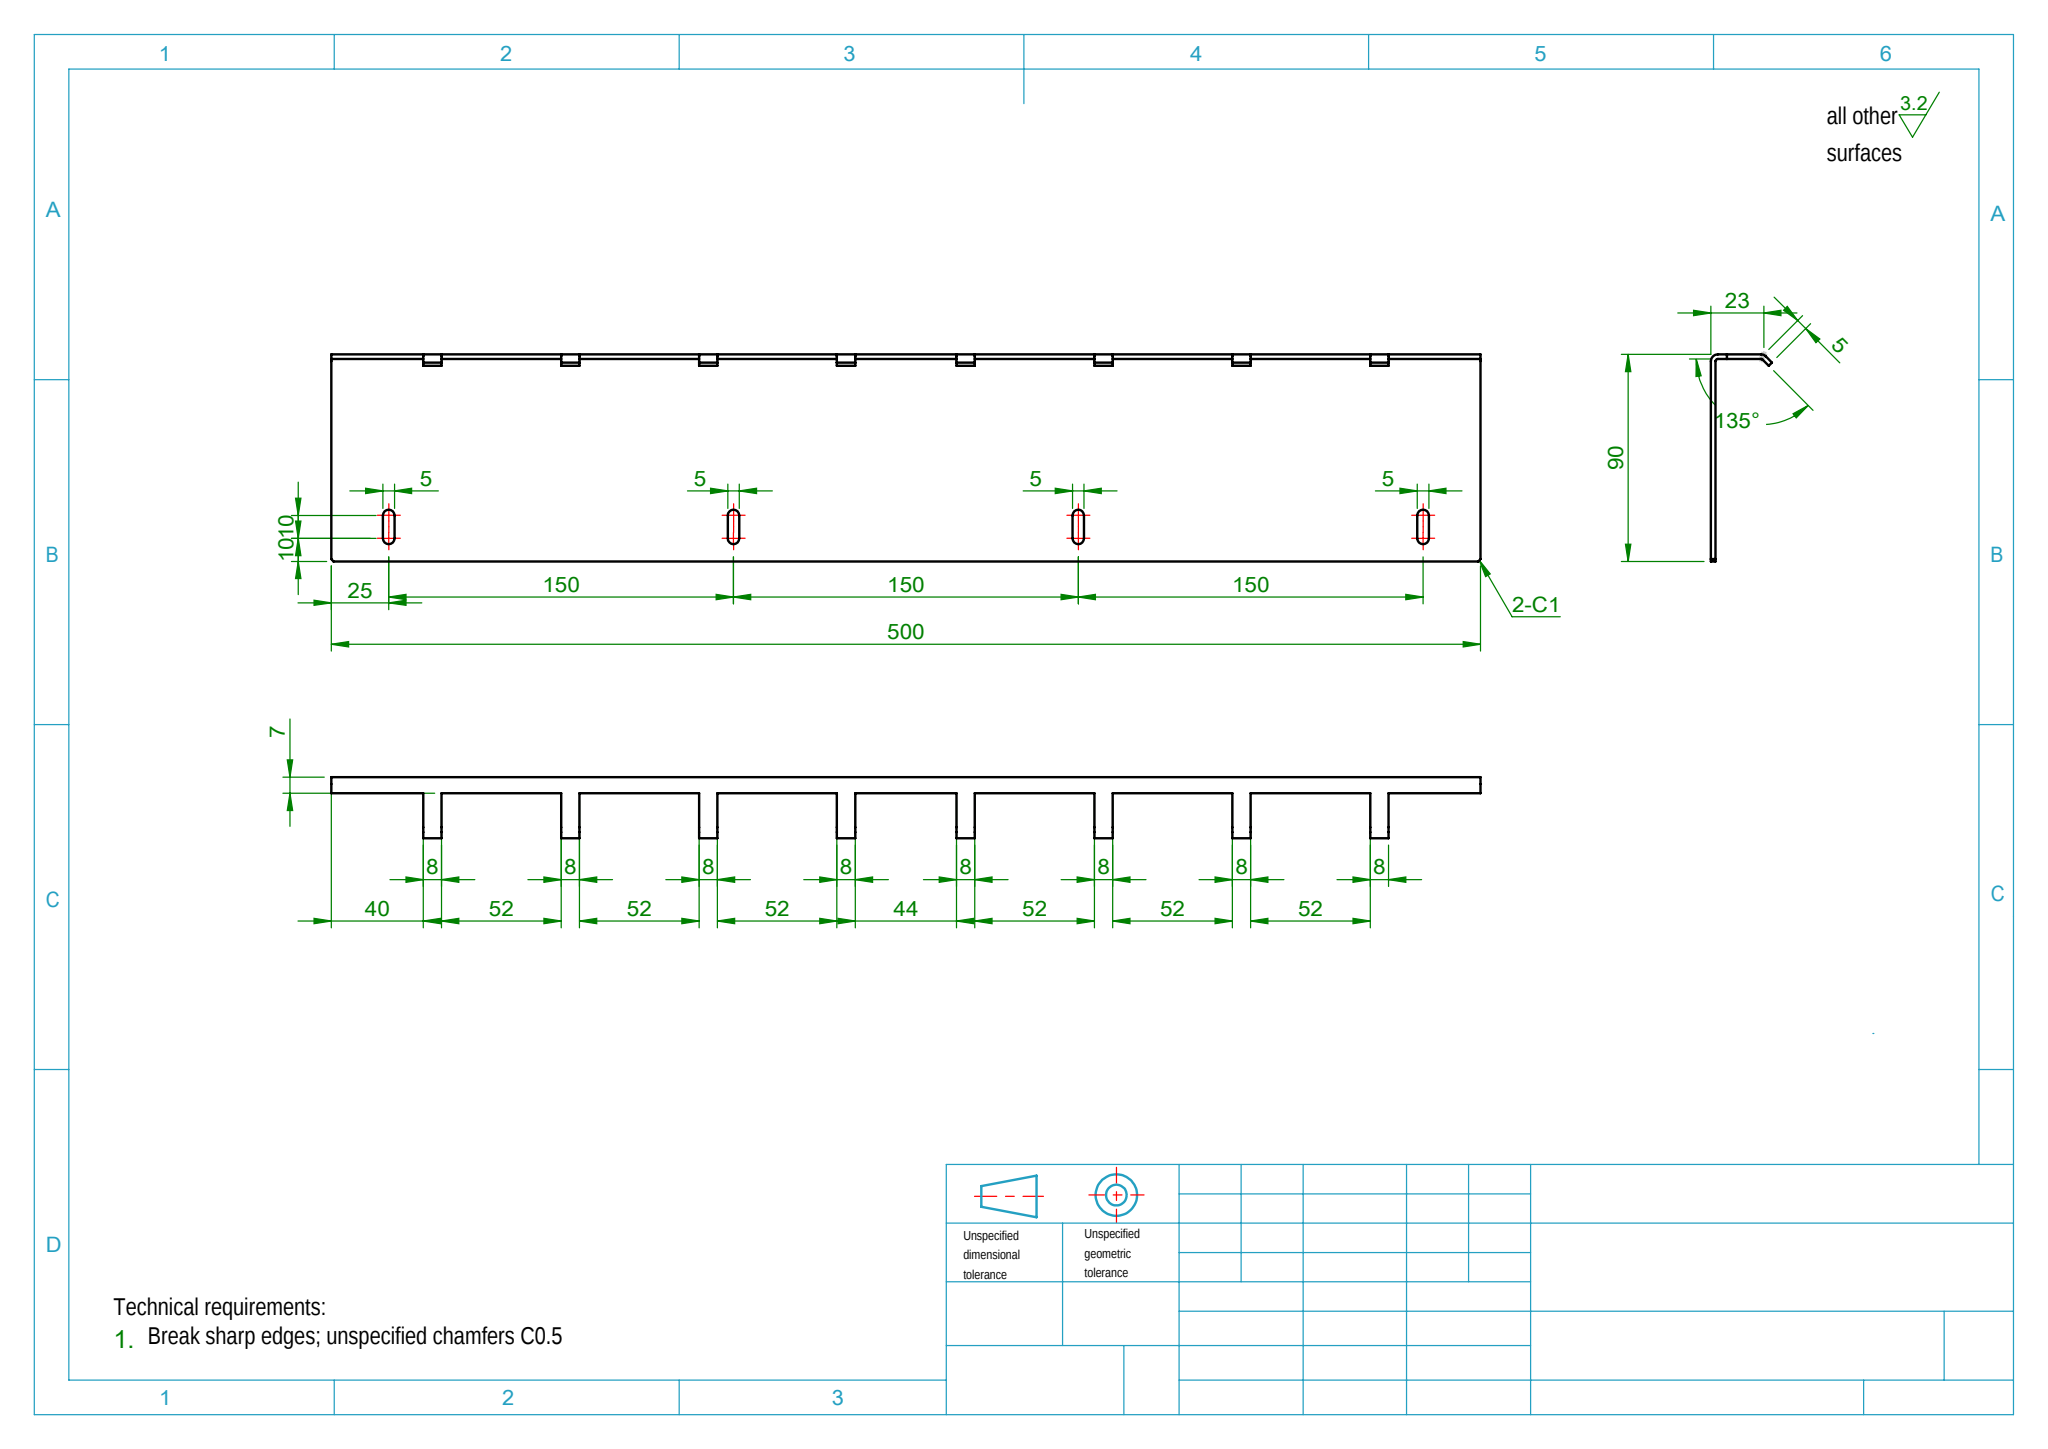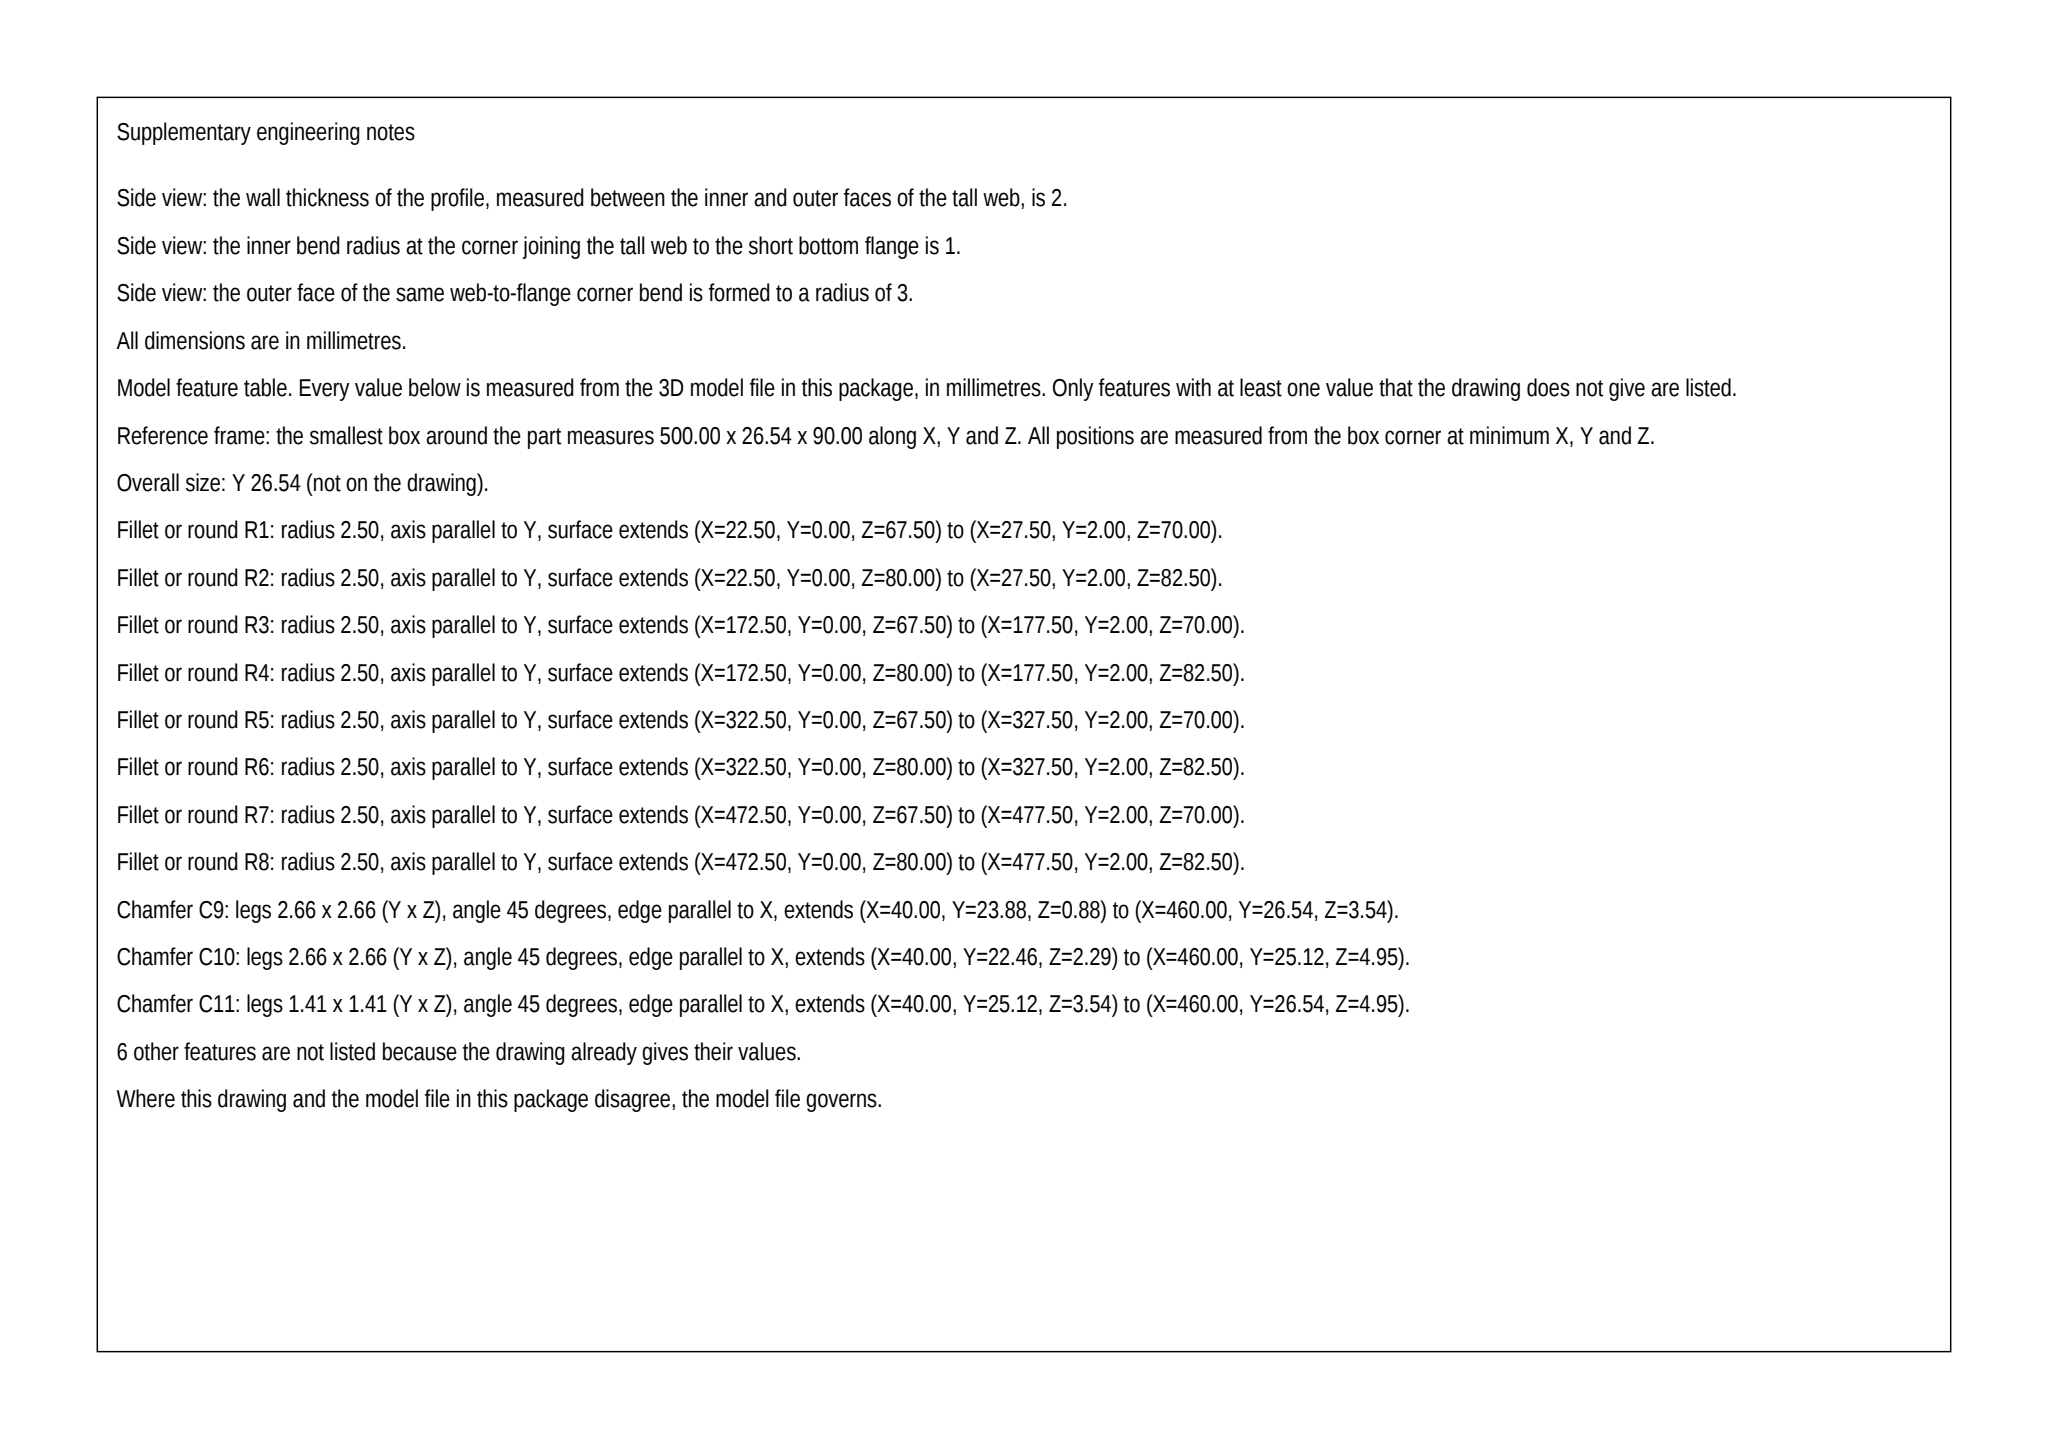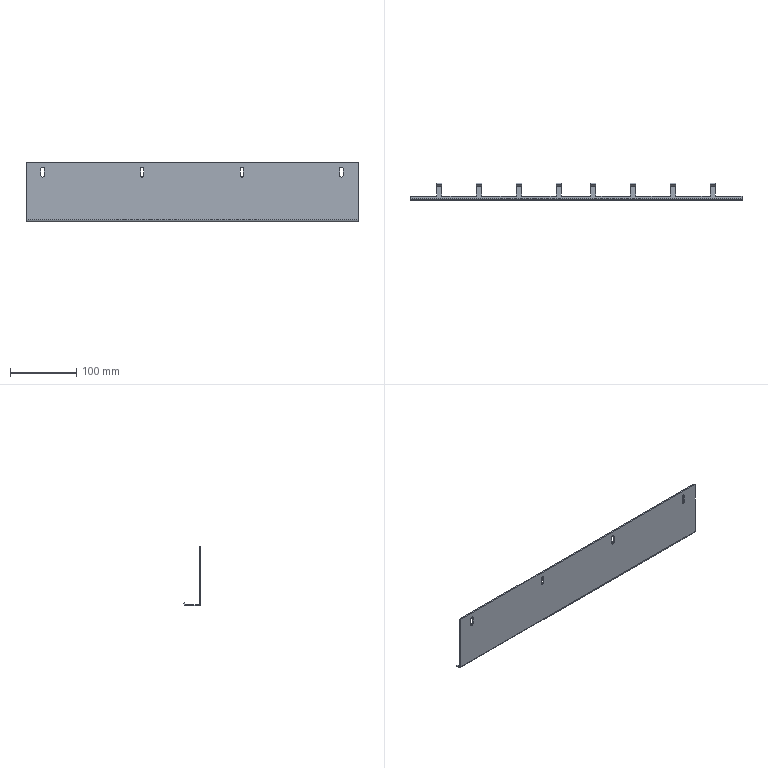Part | SolidWorks | mm | 1 solid | 132 faces | box 500 x 26.54 x 90 mm | volume 96153 mm3 | plane 102 | cylinder 30 | commonest cylinder face diameters 5 x12 6 x9 2 x9